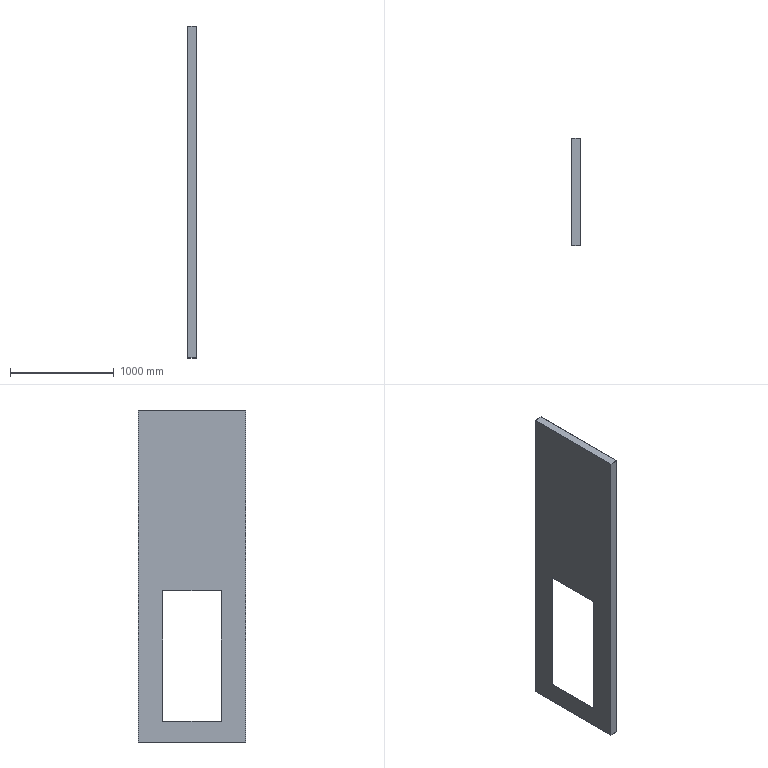Component | NX | DS2 | 1 solid | 19 faces | volume 5025042 mm3 | plane 19